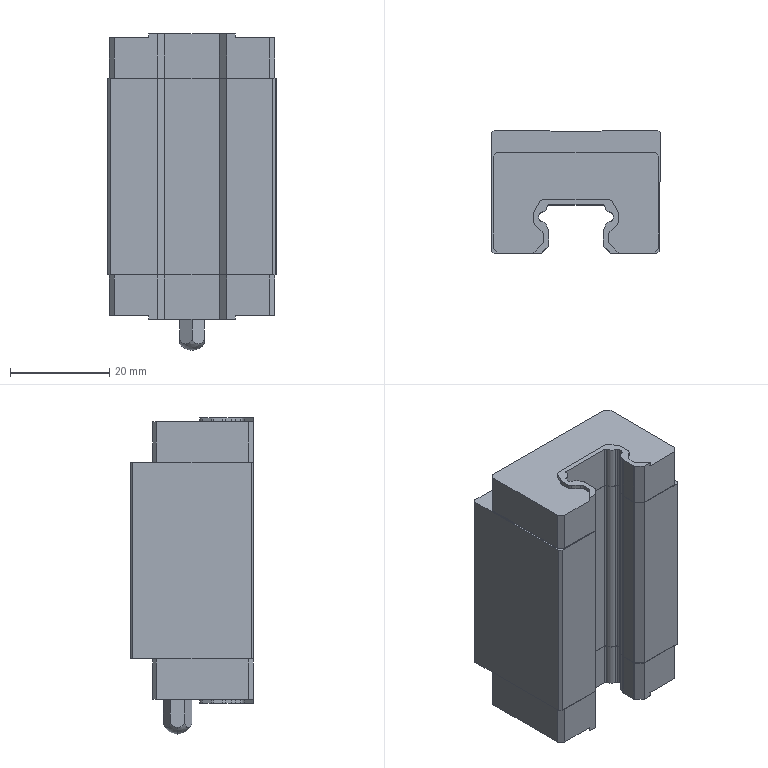Component | SolidWorks | F-YBC_SHR28_R_b-2 | 1 solid | 278 faces | box 34 x 24.8 x 63.7 mm | volume 37331 mm3 | plane 152 | cylinder 108 | cone 16 | sphere 2 | commonest cylinder face diameters 0.6 x36 0.7 x24 2 x20 2.862 x12 3.242 x8 2.962 x8
build123d program:
from build123d import *

# Parameters (mm, degrees)
BOSS_EXTRUDE1_DEPTH      = 19.75
BOSS_EXTRUDE1_DEPTH_BACK = 19.75
BOSS_EXTRUDE2_DEPTH      = 27.95
BOSS_EXTRUDE2_DEPTH_BACK = 27.95
SKETCH4_R                = 3.5
CUT_EXTRUDE1_DEPTH       = 7
BOSS_EXTRUDE3_DEPTH      = 0.8
BOSS_EXTRUDE4_START      = -0.8
BOSS_EXTRUDE4_DEPTH      = 0.8
CUT_EXTRUDE2_DEPTH       = 19.75
CUT_EXTRUDE2_DEPTH_BACK  = 19.75
CUT_EXTRUDE3_DEPTH       = 19.75
CUT_EXTRUDE4_START       = -19.75
CUT_EXTRUDE4_DEPTH       = 19.75
LPATTERN1_COUNT          = 2
LPATTERN1_PITCH          = 26
LPATTERN1_COUNT_DIR2     = 2
LPATTERN1_PITCH_DIR2     = 26
SKETCH12_W               = 36
SKETCH12_H               = 28
CUT_EXTRUDE5_DEPTH       = 0.05
SKETCH13_W               = 36
SKETCH13_H               = 28
CUT_EXTRUDE6_DEPTH       = 0.05
CUT_EXTRUDE7_DEPTH       = 0.05
CUT_EXTRUDE8_START       = -0.05
CUT_EXTRUDE8_DEPTH       = 0.05


with BuildPart() as part:
    # Sketch1 → Boss-Extrude1 (new, two sides: drawn at the far end of the back side and taken through both)
    with BuildSketch(Plane.XY.offset(-BOSS_EXTRUDE1_DEPTH_BACK)):
        Polygon((-17, 17.8), (-16.75, 17.336), (-16.75, 3.7), (-16.25, 3.2), (16.5, 3.2), (17, 3.7), (17, 27.5), (16.5, 28), (5.5, 28), (4.993, 27.7), (-4.993, 27.7), (-5.5, 28), (-16.5, 28), (-17, 27.5), align=None)
    extrude(amount=BOSS_EXTRUDE1_DEPTH + BOSS_EXTRUDE1_DEPTH_BACK)

    # Sketch2 → Boss-Extrude2 (add, two sides: drawn at the far end of the back side and taken through both)
    with BuildSketch(Plane.XY.offset(-BOSS_EXTRUDE2_DEPTH_BACK)):
        Polygon((-16.7, 4.25), (-15.7, 3.25), (15.7, 3.25), (16.7, 4.25), (16.7, 22.75), (15.95, 23.5), (-15.95, 23.5), (-16.7, 22.75), align=None)
    extrude(amount=BOSS_EXTRUDE2_DEPTH + BOSS_EXTRUDE2_DEPTH_BACK)

    # Sketch3 → Revolve1 (revolve)
    with BuildSketch(Plane(origin=(0, 18.5, 0), x_dir=(1, 0, 0), z_dir=(0, 1, 0))):
        with BuildLine():
            Line((-3, -31.95), (-3, -27.95))
            Line((-3, -27.95), (0, -27.95))
            Line((0, -27.95), (0, -34.95))
            ThreePointArc((0, -34.95), (-2.121, -34.071), (-3, -31.95))
        make_face()
    revolve(axis=Axis((0, 18.5, 27.95), (0, 0, 1)))

    # Sketch4 → Cut-Extrude1 (cut)
    with BuildSketch(Plane.XY.offset(27.95)):
        with Locations((0, 18.5)):
            Circle(SKETCH4_R)
        Polygon((-2.5, 19.943), (-2.5, 17.057), (0, 15.613), (2.5, 17.057), (2.5, 19.943), (0, 21.387), align=None, mode=Mode.SUBTRACT)
    extrude(amount=CUT_EXTRUDE1_DEPTH, mode=Mode.SUBTRACT)

    # Sketch5 → Boss-Extrude3 (add)
    with BuildSketch(Plane.XY.offset(27.95)):
        with BuildLine():
            Line((-8.664, 3.25), (8.664, 3.25))
            Line((8.664, 3.25), (6.793, 5.122))
            ThreePointArc((6.793, 5.122), (6.576, 5.446), (6.5, 5.829))
            Line((6.5, 5.829), (6.5, 6.855))
            ThreePointArc((6.5, 6.855), (6.587, 7.263), (6.833, 7.601))
            Line((6.833, 7.601), (8.167, 8.793))
            ThreePointArc((8.167, 8.793), (8.413, 9.13), (8.5, 9.539))
            Line((8.5, 9.539), (8.5, 11.248))
            ThreePointArc((8.5, 11.248), (8.468, 11.5), (8.373, 11.736))
            Line((8.373, 11.736), (7.391, 13.489))
            ThreePointArc((7.391, 13.489), (7.025, 13.863), (6.519, 14))
            Line((6.519, 14), (-6.519, 14))
            ThreePointArc((-6.519, 14), (-7.025, 13.863), (-7.391, 13.489))
            Line((-7.391, 13.489), (-8.373, 11.736))
            ThreePointArc((-8.373, 11.736), (-8.468, 11.5), (-8.5, 11.248))
            Line((-8.5, 11.248), (-8.5, 9.539))
            ThreePointArc((-8.5, 9.539), (-8.413, 9.13), (-8.167, 8.793))
            Line((-8.167, 8.793), (-6.833, 7.601))
            ThreePointArc((-6.833, 7.601), (-6.587, 7.263), (-6.5, 6.855))
            Line((-6.5, 6.855), (-6.5, 5.829))
            ThreePointArc((-6.5, 5.829), (-6.576, 5.446), (-6.793, 5.122))
            Line((-6.793, 5.122), (-8.664, 3.25))
        make_face()
    extrude(amount=BOSS_EXTRUDE3_DEPTH)

    # Sketch6 → Boss-Extrude4 (add)
    with BuildSketch(Plane.XY.offset(-27.95).offset(BOSS_EXTRUDE4_START)):
        with BuildLine():
            Line((-8.664, 3.25), (8.664, 3.25))
            Line((8.664, 3.25), (6.793, 5.122))
            ThreePointArc((6.793, 5.122), (6.576, 5.446), (6.5, 5.829))
            Line((6.5, 5.829), (6.5, 6.855))
            ThreePointArc((6.5, 6.855), (6.587, 7.263), (6.833, 7.601))
            Line((6.833, 7.601), (8.167, 8.793))
            ThreePointArc((8.167, 8.793), (8.413, 9.13), (8.5, 9.539))
            Line((8.5, 9.539), (8.5, 11.248))
            ThreePointArc((8.5, 11.248), (8.468, 11.5), (8.373, 11.736))
            Line((8.373, 11.736), (7.391, 13.489))
            ThreePointArc((7.391, 13.489), (7.025, 13.863), (6.519, 14))
            Line((6.519, 14), (-6.519, 14))
            ThreePointArc((-6.519, 14), (-7.025, 13.863), (-7.391, 13.489))
            Line((-7.391, 13.489), (-8.373, 11.736))
            ThreePointArc((-8.373, 11.736), (-8.468, 11.5), (-8.5, 11.248))
            Line((-8.5, 11.248), (-8.5, 9.539))
            ThreePointArc((-8.5, 9.539), (-8.413, 9.13), (-8.167, 8.793))
            Line((-8.167, 8.793), (-6.833, 7.601))
            ThreePointArc((-6.833, 7.601), (-6.587, 7.263), (-6.5, 6.855))
            Line((-6.5, 6.855), (-6.5, 5.829))
            ThreePointArc((-6.5, 5.829), (-6.576, 5.446), (-6.793, 5.122))
            Line((-6.793, 5.122), (-8.664, 3.25))
        make_face()
    extrude(amount=BOSS_EXTRUDE4_DEPTH)

    # Sketch7 → Cut-Extrude2 (cut, two sides: drawn at the far end of the back side and taken through both)
    with BuildSketch(Plane.XY.offset(-CUT_EXTRUDE2_DEPTH_BACK)):
        with BuildLine():
            Line((-7.5, 2.576), (-7.5, 0.5))
            Line((-7.5, 0.5), (-7, 0))
            Line((-7, 0), (7, 0))
            Line((7, 0), (7.5, 0.5))
            Line((7.5, 0.5), (7.5, 2.576))
            ThreePointArc((7.5, 2.576), (7.477, 2.691), (7.412, 2.788))
            Line((7.412, 2.788), (5.588, 4.612))
            ThreePointArc((5.588, 4.612), (5.523, 4.709), (5.5, 4.824))
            Line((5.5, 4.824), (5.5, 7.797))
            ThreePointArc((5.5, 7.797), (5.523, 7.912), (5.588, 8.009))
            Line((5.588, 8.009), (5.702, 8.123))
            ThreePointArc((5.702, 8.123), (5.763, 8.211), (5.789, 8.315))
            ThreePointArc((5.789, 8.315), (6.174, 9.2), (7.033, 9.64))
            ThreePointArc((7.033, 9.64), (7.171, 9.695), (7.266, 9.811))
            Line((7.266, 9.811), (7.5, 10.313))
            Line((7.5, 10.313), (7.5, 10.787))
            Line((7.5, 10.787), (7.265, 11.29))
            ThreePointArc((7.265, 11.29), (7.171, 11.406), (7.032, 11.461))
            ThreePointArc((7.032, 11.461), (6.192, 11.881), (5.794, 12.731))
            ThreePointArc((5.794, 12.731), (5.696, 12.923), (5.495, 13))
            Line((5.495, 13), (-5.495, 13))
            ThreePointArc((-5.495, 13), (-5.696, 12.923), (-5.794, 12.731))
            ThreePointArc((-5.794, 12.731), (-6.192, 11.881), (-7.032, 11.461))
            ThreePointArc((-7.032, 11.461), (-7.171, 11.406), (-7.265, 11.29))
            Line((-7.265, 11.29), (-7.5, 10.787))
            Line((-7.5, 10.787), (-7.5, 10.313))
            Line((-7.5, 10.313), (-7.266, 9.811))
            ThreePointArc((-7.266, 9.811), (-7.171, 9.695), (-7.033, 9.64))
            ThreePointArc((-7.033, 9.64), (-6.174, 9.2), (-5.789, 8.315))
            ThreePointArc((-5.789, 8.315), (-5.763, 8.211), (-5.702, 8.123))
            Line((-5.702, 8.123), (-5.588, 8.009))
            ThreePointArc((-5.588, 8.009), (-5.523, 7.912), (-5.5, 7.797))
            Line((-5.5, 7.797), (-5.5, 4.824))
            ThreePointArc((-5.5, 4.824), (-5.523, 4.709), (-5.588, 4.612))
            Line((-5.588, 4.612), (-7.412, 2.788))
            ThreePointArc((-7.412, 2.788), (-7.477, 2.691), (-7.5, 2.576))
        make_face()
    extrude(amount=CUT_EXTRUDE2_DEPTH + CUT_EXTRUDE2_DEPTH_BACK, mode=Mode.SUBTRACT)

    # Sketch8 → Cut-Extrude3 (cut)
    with BuildSketch(Plane.XY.offset(19.75)):
        with BuildLine():
            Line((-7.5, 2.576), (-7.5, 0.5))
            Line((-7.5, 0.5), (-7, 0))
            Line((-7, 0), (7, 0))
            Line((7, 0), (7.5, 0.5))
            Line((7.5, 0.5), (7.5, 2.576))
            ThreePointArc((7.5, 2.576), (7.477, 2.691), (7.412, 2.788))
            Line((7.412, 2.788), (5.588, 4.612))
            ThreePointArc((5.588, 4.612), (5.523, 4.709), (5.5, 4.824))
            Line((5.5, 4.824), (5.5, 7.797))
            ThreePointArc((5.5, 7.797), (5.523, 7.912), (5.588, 8.009))
            Line((5.588, 8.009), (5.702, 8.123))
            ThreePointArc((5.702, 8.123), (5.763, 8.211), (5.789, 8.315))
            ThreePointArc((5.789, 8.315), (6.174, 9.2), (7.033, 9.64))
            ThreePointArc((7.033, 9.64), (7.171, 9.695), (7.266, 9.811))
            Line((7.266, 9.811), (7.5, 10.313))
            Line((7.5, 10.313), (7.5, 10.787))
            Line((7.5, 10.787), (7.265, 11.29))
            ThreePointArc((7.265, 11.29), (7.171, 11.406), (7.032, 11.461))
            ThreePointArc((7.032, 11.461), (6.192, 11.881), (5.794, 12.731))
            ThreePointArc((5.794, 12.731), (5.696, 12.923), (5.495, 13))
            Line((5.495, 13), (-5.495, 13))
            ThreePointArc((-5.495, 13), (-5.696, 12.923), (-5.794, 12.731))
            ThreePointArc((-5.794, 12.731), (-6.192, 11.881), (-7.032, 11.461))
            ThreePointArc((-7.032, 11.461), (-7.171, 11.406), (-7.265, 11.29))
            Line((-7.265, 11.29), (-7.5, 10.787))
            Line((-7.5, 10.787), (-7.5, 10.313))
            Line((-7.5, 10.313), (-7.266, 9.811))
            ThreePointArc((-7.266, 9.811), (-7.171, 9.695), (-7.033, 9.64))
            ThreePointArc((-7.033, 9.64), (-6.174, 9.2), (-5.789, 8.315))
            ThreePointArc((-5.789, 8.315), (-5.763, 8.211), (-5.702, 8.123))
            Line((-5.702, 8.123), (-5.588, 8.009))
            ThreePointArc((-5.588, 8.009), (-5.523, 7.912), (-5.5, 7.797))
            Line((-5.5, 7.797), (-5.5, 4.824))
            ThreePointArc((-5.5, 4.824), (-5.523, 4.709), (-5.588, 4.612))
            Line((-5.588, 4.612), (-7.412, 2.788))
            ThreePointArc((-7.412, 2.788), (-7.477, 2.691), (-7.5, 2.576))
        make_face()
    extrude(amount=CUT_EXTRUDE3_DEPTH, mode=Mode.SUBTRACT)

    # Sketch9 → Cut-Extrude4 (cut)
    with BuildSketch(Plane.XY.offset(-19.75).offset(CUT_EXTRUDE4_START)):
        with BuildLine():
            Line((-7.5, 2.576), (-7.5, 0.5))
            Line((-7.5, 0.5), (-7, 0))
            Line((-7, 0), (7, 0))
            Line((7, 0), (7.5, 0.5))
            Line((7.5, 0.5), (7.5, 2.576))
            ThreePointArc((7.5, 2.576), (7.477, 2.691), (7.412, 2.788))
            Line((7.412, 2.788), (5.588, 4.612))
            ThreePointArc((5.588, 4.612), (5.523, 4.709), (5.5, 4.824))
            Line((5.5, 4.824), (5.5, 7.797))
            ThreePointArc((5.5, 7.797), (5.523, 7.912), (5.588, 8.009))
            Line((5.588, 8.009), (5.702, 8.123))
            ThreePointArc((5.702, 8.123), (5.763, 8.211), (5.789, 8.315))
            ThreePointArc((5.789, 8.315), (6.174, 9.2), (7.033, 9.64))
            ThreePointArc((7.033, 9.64), (7.171, 9.695), (7.266, 9.811))
            Line((7.266, 9.811), (7.5, 10.313))
            Line((7.5, 10.313), (7.5, 10.787))
            Line((7.5, 10.787), (7.265, 11.29))
            ThreePointArc((7.265, 11.29), (7.171, 11.406), (7.032, 11.461))
            ThreePointArc((7.032, 11.461), (6.192, 11.881), (5.794, 12.731))
            ThreePointArc((5.794, 12.731), (5.696, 12.923), (5.495, 13))
            Line((5.495, 13), (-5.495, 13))
            ThreePointArc((-5.495, 13), (-5.696, 12.923), (-5.794, 12.731))
            ThreePointArc((-5.794, 12.731), (-6.192, 11.881), (-7.032, 11.461))
            ThreePointArc((-7.032, 11.461), (-7.171, 11.406), (-7.265, 11.29))
            Line((-7.265, 11.29), (-7.5, 10.787))
            Line((-7.5, 10.787), (-7.5, 10.313))
            Line((-7.5, 10.313), (-7.266, 9.811))
            ThreePointArc((-7.266, 9.811), (-7.171, 9.695), (-7.033, 9.64))
            ThreePointArc((-7.033, 9.64), (-6.174, 9.2), (-5.789, 8.315))
            ThreePointArc((-5.789, 8.315), (-5.763, 8.211), (-5.702, 8.123))
            Line((-5.702, 8.123), (-5.588, 8.009))
            ThreePointArc((-5.588, 8.009), (-5.523, 7.912), (-5.5, 7.797))
            Line((-5.5, 7.797), (-5.5, 4.824))
            ThreePointArc((-5.5, 4.824), (-5.523, 4.709), (-5.588, 4.612))
            Line((-5.588, 4.612), (-7.412, 2.788))
            ThreePointArc((-7.412, 2.788), (-7.477, 2.691), (-7.5, 2.576))
        make_face()
    extrude(amount=CUT_EXTRUDE4_DEPTH, mode=Mode.SUBTRACT)

    # Sketch10 → Cut-Revolve1 (revolve, cut)
    with BuildSketch(Plane.XY.offset(13), mode=Mode.PRIVATE) as cut_revolve1_sk:
        Polygon((-13, 19.964), (-14.621, 20.9), (-14.621, 27.621), (-15, 28), (-13, 28), align=None)
    cut_revolve1 = revolve(cut_revolve1_sk.sketch.rotate(Axis((-13, 28, 13), (0, -1, 0)), 90), axis=Axis((-13, 28, 13), (0, -1, 0)), mode=Mode.SUBTRACT)

    # LPattern1: Cut-Revolve1 2 × 2
    with Locations(*[(i * LPATTERN1_PITCH, 0, -j * LPATTERN1_PITCH_DIR2) for i in range(LPATTERN1_COUNT) for j in range(LPATTERN1_COUNT_DIR2) if (i, j) != (0, 0)]):
        add(cut_revolve1, mode=Mode.SUBTRACT)

    # Sketch12 → Cut-Extrude5 (cut)
    with BuildSketch(Plane.XY.offset(19.75)):
        with Locations((0, 16)):
            Rectangle(SKETCH12_W, SKETCH12_H)
        Polygon((-16.65, 22.729), (-16.65, 4.271), (-15.679, 3.3), (15.679, 3.3), (16.65, 4.271), (16.65, 22.729), (15.929, 23.45), (-15.929, 23.45), align=None, mode=Mode.SUBTRACT)
    extrude(amount=CUT_EXTRUDE5_DEPTH, mode=Mode.SUBTRACT)

    # Sketch13 → Cut-Extrude6 (cut)
    with BuildSketch(Plane.XY.offset(-19.75)):
        with Locations((0, 16)):
            Rectangle(SKETCH13_W, SKETCH13_H)
        Polygon((-16.65, 22.729), (-16.65, 4.271), (-15.679, 3.3), (15.679, 3.3), (16.65, 4.271), (16.65, 22.729), (15.929, 23.45), (-15.929, 23.45), align=None, mode=Mode.SUBTRACT)
    extrude(amount=-CUT_EXTRUDE6_DEPTH, mode=Mode.SUBTRACT)

    # Sketch14 → Cut-Extrude7 (cut)
    with BuildSketch(Plane.XY.offset(19.75)):
        with BuildLine():
            Line((-7.55, 0.5), (-7.05, 0))
            Line((-7.05, 0), (7.05, 0))
            Line((7.05, 0), (7.55, 0.5))
            Line((7.55, 0.5), (7.55, 2.602))
            ThreePointArc((7.55, 2.602), (7.523, 2.736), (7.448, 2.849))
            Line((7.448, 2.849), (5.652, 4.648))
            ThreePointArc((5.652, 4.648), (5.577, 4.761), (5.55, 4.895))
            Line((5.55, 4.895), (5.55, 7.776))
            ThreePointArc((5.55, 7.776), (5.577, 7.91), (5.652, 8.023))
            Line((5.652, 8.023), (5.689, 8.06))
            ThreePointArc((5.689, 8.06), (5.759, 8.162), (5.79, 8.281))
            ThreePointArc((5.79, 8.281), (6.179, 9.176), (7.039, 9.634))
            ThreePointArc((7.039, 9.634), (7.196, 9.7), (7.303, 9.832))
            Line((7.303, 9.832), (7.55, 10.363))
            Line((7.55, 10.363), (7.55, 10.887))
            Line((7.55, 10.887), (7.377, 11.259))
            ThreePointArc((7.377, 11.259), (7.264, 11.395), (7.099, 11.459))
            ThreePointArc((7.099, 11.459), (6.226, 11.876), (5.798, 12.744))
            ThreePointArc((5.798, 12.744), (5.682, 12.963), (5.451, 13.05))
            Line((5.451, 13.05), (-5.451, 13.05))
            ThreePointArc((-5.451, 13.05), (-5.682, 12.963), (-5.798, 12.744))
            ThreePointArc((-5.798, 12.744), (-6.226, 11.876), (-7.099, 11.459))
            ThreePointArc((-7.099, 11.459), (-7.264, 11.395), (-7.377, 11.259))
            Line((-7.377, 11.259), (-7.55, 10.887))
            Line((-7.55, 10.887), (-7.55, 10.363))
            Line((-7.55, 10.363), (-7.303, 9.832))
            ThreePointArc((-7.303, 9.832), (-7.196, 9.7), (-7.039, 9.634))
            ThreePointArc((-7.039, 9.634), (-6.179, 9.176), (-5.79, 8.281))
            ThreePointArc((-5.79, 8.281), (-5.759, 8.162), (-5.689, 8.06))
            Line((-5.689, 8.06), (-5.652, 8.023))
            ThreePointArc((-5.652, 8.023), (-5.577, 7.91), (-5.55, 7.776))
            Line((-5.55, 7.776), (-5.55, 4.895))
            ThreePointArc((-5.55, 4.895), (-5.577, 4.761), (-5.652, 4.648))
            Line((-5.652, 4.648), (-7.448, 2.849))
            ThreePointArc((-7.448, 2.849), (-7.523, 2.736), (-7.55, 2.602))
            Line((-7.55, 2.602), (-7.55, 0.5))
        make_face()
    extrude(amount=CUT_EXTRUDE7_DEPTH, mode=Mode.SUBTRACT)

    # Sketch15 → Cut-Extrude8 (cut)
    with BuildSketch(Plane.XY.offset(-19.75).offset(CUT_EXTRUDE8_START)):
        with BuildLine():
            Line((-7.55, 0.5), (-7.05, 0))
            Line((-7.05, 0), (7.05, 0))
            Line((7.05, 0), (7.55, 0.5))
            Line((7.55, 0.5), (7.55, 2.602))
            ThreePointArc((7.55, 2.602), (7.523, 2.736), (7.448, 2.849))
            Line((7.448, 2.849), (5.652, 4.648))
            ThreePointArc((5.652, 4.648), (5.577, 4.761), (5.55, 4.895))
            Line((5.55, 4.895), (5.55, 7.776))
            ThreePointArc((5.55, 7.776), (5.577, 7.91), (5.652, 8.023))
            Line((5.652, 8.023), (5.689, 8.06))
            ThreePointArc((5.689, 8.06), (5.759, 8.162), (5.79, 8.281))
            ThreePointArc((5.79, 8.281), (6.179, 9.176), (7.039, 9.634))
            ThreePointArc((7.039, 9.634), (7.196, 9.7), (7.303, 9.832))
            Line((7.303, 9.832), (7.55, 10.363))
            Line((7.55, 10.363), (7.55, 10.887))
            Line((7.55, 10.887), (7.377, 11.259))
            ThreePointArc((7.377, 11.259), (7.264, 11.395), (7.099, 11.459))
            ThreePointArc((7.099, 11.459), (6.226, 11.876), (5.798, 12.744))
            ThreePointArc((5.798, 12.744), (5.682, 12.963), (5.451, 13.05))
            Line((5.451, 13.05), (-5.451, 13.05))
            ThreePointArc((-5.451, 13.05), (-5.682, 12.963), (-5.798, 12.744))
            ThreePointArc((-5.798, 12.744), (-6.226, 11.876), (-7.099, 11.459))
            ThreePointArc((-7.099, 11.459), (-7.264, 11.395), (-7.377, 11.259))
            Line((-7.377, 11.259), (-7.55, 10.887))
            Line((-7.55, 10.887), (-7.55, 10.363))
            Line((-7.55, 10.363), (-7.303, 9.832))
            ThreePointArc((-7.303, 9.832), (-7.196, 9.7), (-7.039, 9.634))
            ThreePointArc((-7.039, 9.634), (-6.179, 9.176), (-5.79, 8.281))
            ThreePointArc((-5.79, 8.281), (-5.759, 8.162), (-5.689, 8.06))
            Line((-5.689, 8.06), (-5.652, 8.023))
            ThreePointArc((-5.652, 8.023), (-5.577, 7.91), (-5.55, 7.776))
            Line((-5.55, 7.776), (-5.55, 4.895))
            ThreePointArc((-5.55, 4.895), (-5.577, 4.761), (-5.652, 4.648))
            Line((-5.652, 4.648), (-7.448, 2.849))
            ThreePointArc((-7.448, 2.849), (-7.523, 2.736), (-7.55, 2.602))
            Line((-7.55, 2.602), (-7.55, 0.5))
        make_face()
    extrude(amount=CUT_EXTRUDE8_DEPTH, mode=Mode.SUBTRACT)


solid = part.part

# Placed as in the assembly
solid = solid.moved(Location((349.305, 292.175, 129.979), (-180, 0, 180)))